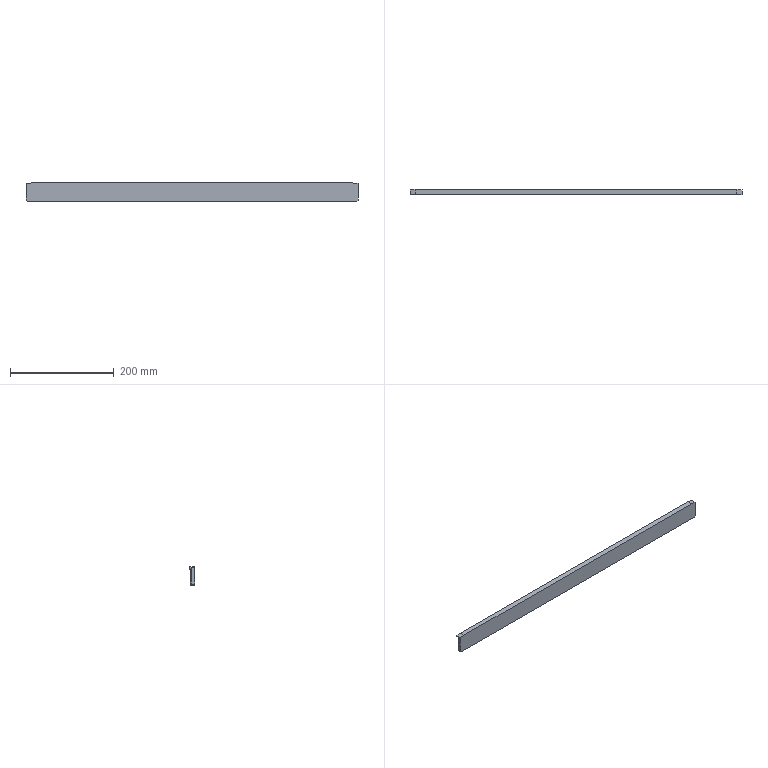Component | SolidWorks | XT-1-04-2-1 | 1 solid | 40 faces | box 640 x 10 x 35 mm | volume 184177 mm3 | plane 20 | cylinder 10 | cone 10 | commonest cylinder face diameters 3.3 x10
STEP:
#1=COLOUR_RGB('',0.7922,0.8196,0.9333);
#2=FILL_AREA_STYLE_COLOUR('',#1);
#3=FILL_AREA_STYLE('',(#2));
#4=SURFACE_STYLE_FILL_AREA(#3);
#5=SURFACE_SIDE_STYLE('',(#4));
#6=SURFACE_STYLE_USAGE(.BOTH.,#5);
#7=PRESENTATION_STYLE_ASSIGNMENT((#6));
#8=CARTESIAN_POINT('',(34.289,4.936,-5.035));
#9=VERTEX_POINT('',#8);
#10=CARTESIAN_POINT('',(34.159,4.936,-5.035));
#11=VERTEX_POINT('',#10);
#12=CARTESIAN_POINT('',(34.224,4.936,-5.035));
#13=DIRECTION('',(0.,0.,-1.));
#14=DIRECTION('',(-1.,0.,0.));
#15=AXIS2_PLACEMENT_3D('',#12,#13,#14);
#16=CIRCLE('',#15,0.06496);
#17=EDGE_CURVE('',#9,#11,#16,.T.);
#18=ORIENTED_EDGE('',*,*,#17,.F.);
#19=CARTESIAN_POINT('',(34.289,4.936,-5.433));
#20=VERTEX_POINT('',#19);
#21=CARTESIAN_POINT('',(34.289,4.936,-5.433));
#22=DIRECTION('',(0.,0.,-1.));
#23=VECTOR('',#22,39.37);
#24=LINE('',#21,#23);
#25=EDGE_CURVE('',#9,#20,#24,.T.);
#26=ORIENTED_EDGE('',*,*,#25,.T.);
#27=CARTESIAN_POINT('',(34.159,4.936,-5.433));
#28=VERTEX_POINT('',#27);
#29=CARTESIAN_POINT('',(34.224,4.936,-5.433));
#30=DIRECTION('',(0.,0.,-1.));
#31=DIRECTION('',(-1.,0.,0.));
#32=AXIS2_PLACEMENT_3D('',#29,#30,#31);
#33=CIRCLE('',#32,0.06496);
#34=EDGE_CURVE('',#20,#28,#33,.T.);
#35=ORIENTED_EDGE('',*,*,#34,.T.);
#36=CARTESIAN_POINT('',(34.159,4.936,-5.433));
#37=DIRECTION('',(0.,0.,-1.));
#38=VECTOR('',#37,39.37);
#39=LINE('',#36,#38);
#40=EDGE_CURVE('',#11,#28,#39,.T.);
#41=ORIENTED_EDGE('',*,*,#40,.F.);
#42=EDGE_LOOP('',(#18,#26,#35,#41));
#43=FACE_OUTER_BOUND('',#42,.T.);
#44=CARTESIAN_POINT('',(34.224,4.936,-5.433));
#45=DIRECTION('',(0.,0.,-1.));
#46=DIRECTION('',(-1.,0.,0.));
#47=AXIS2_PLACEMENT_3D('',#44,#45,#46);
#48=CYLINDRICAL_SURFACE('',#47,0.06496);
#49=ADVANCED_FACE('',(#43),#48,.F.);
#50=CARTESIAN_POINT('',(34.224,4.936,-4.996));
#51=VERTEX_POINT('',#50);
#52=CARTESIAN_POINT('',(34.159,4.936,-5.035));
#53=DIRECTION('',(-0.8572,0.,-0.515));
#54=VECTOR('',#53,39.37);
#55=LINE('',#52,#54);
#56=EDGE_CURVE('',#51,#11,#55,.T.);
#57=ORIENTED_EDGE('',*,*,#56,.F.);
#58=CARTESIAN_POINT('',(34.289,4.936,-5.035));
#59=DIRECTION('',(0.8572,0.,-0.515));
#60=VECTOR('',#59,39.37);
#61=LINE('',#58,#60);
#62=EDGE_CURVE('',#51,#9,#61,.T.);
#63=ORIENTED_EDGE('',*,*,#62,.T.);
#64=ORIENTED_EDGE('',*,*,#17,.T.);
#65=EDGE_LOOP('',(#57,#63,#64));
#66=FACE_OUTER_BOUND('',#65,.T.);
#67=CARTESIAN_POINT('',(34.224,4.936,-5.035));
#68=DIRECTION('',(0.,0.,-1.));
#69=DIRECTION('',(-1.,0.,0.));
#70=AXIS2_PLACEMENT_3D('',#67,#68,#69);
#71=CONICAL_SURFACE('',#70,0.06496,1.03);
#72=ADVANCED_FACE('',(#66),#71,.F.);
#73=CARTESIAN_POINT('',(28.777,4.936,-5.035));
#74=VERTEX_POINT('',#73);
#75=CARTESIAN_POINT('',(28.647,4.936,-5.035));
#76=VERTEX_POINT('',#75);
#77=CARTESIAN_POINT('',(28.712,4.936,-5.035));
#78=DIRECTION('',(0.,0.,-1.));
#79=DIRECTION('',(-1.,0.,0.));
#80=AXIS2_PLACEMENT_3D('',#77,#78,#79);
#81=CIRCLE('',#80,0.06496);
#82=EDGE_CURVE('',#74,#76,#81,.T.);
#83=ORIENTED_EDGE('',*,*,#82,.F.);
#84=CARTESIAN_POINT('',(28.777,4.936,-5.433));
#85=VERTEX_POINT('',#84);
#86=CARTESIAN_POINT('',(28.777,4.936,-5.433));
#87=DIRECTION('',(0.,0.,-1.));
#88=VECTOR('',#87,39.37);
#89=LINE('',#86,#88);
#90=EDGE_CURVE('',#74,#85,#89,.T.);
#91=ORIENTED_EDGE('',*,*,#90,.T.);
#92=CARTESIAN_POINT('',(28.647,4.936,-5.433));
#93=VERTEX_POINT('',#92);
#94=CARTESIAN_POINT('',(28.712,4.936,-5.433));
#95=DIRECTION('',(0.,0.,-1.));
#96=DIRECTION('',(-1.,0.,0.));
#97=AXIS2_PLACEMENT_3D('',#94,#95,#96);
#98=CIRCLE('',#97,0.06496);
#99=EDGE_CURVE('',#85,#93,#98,.T.);
#100=ORIENTED_EDGE('',*,*,#99,.T.);
#101=CARTESIAN_POINT('',(28.647,4.936,-5.433));
#102=DIRECTION('',(0.,0.,-1.));
#103=VECTOR('',#102,39.37);
#104=LINE('',#101,#103);
#105=EDGE_CURVE('',#76,#93,#104,.T.);
#106=ORIENTED_EDGE('',*,*,#105,.F.);
#107=EDGE_LOOP('',(#83,#91,#100,#106));
#108=FACE_OUTER_BOUND('',#107,.T.);
#109=CARTESIAN_POINT('',(28.712,4.936,-5.433));
#110=DIRECTION('',(0.,0.,-1.));
#111=DIRECTION('',(-1.,0.,0.));
#112=AXIS2_PLACEMENT_3D('',#109,#110,#111);
#113=CYLINDRICAL_SURFACE('',#112,0.06496);
#114=ADVANCED_FACE('',(#108),#113,.F.);
#115=CARTESIAN_POINT('',(28.712,4.936,-4.996));
#116=VERTEX_POINT('',#115);
#117=CARTESIAN_POINT('',(28.647,4.936,-5.035));
#118=DIRECTION('',(-0.8572,0.,-0.515));
#119=VECTOR('',#118,39.37);
#120=LINE('',#117,#119);
#121=EDGE_CURVE('',#116,#76,#120,.T.);
#122=ORIENTED_EDGE('',*,*,#121,.F.);
#123=CARTESIAN_POINT('',(28.777,4.936,-5.035));
#124=DIRECTION('',(0.8572,0.,-0.515));
#125=VECTOR('',#124,39.37);
#126=LINE('',#123,#125);
#127=EDGE_CURVE('',#116,#74,#126,.T.);
#128=ORIENTED_EDGE('',*,*,#127,.T.);
#129=ORIENTED_EDGE('',*,*,#82,.T.);
#130=EDGE_LOOP('',(#122,#128,#129));
#131=FACE_OUTER_BOUND('',#130,.T.);
#132=CARTESIAN_POINT('',(28.712,4.936,-5.035));
#133=DIRECTION('',(0.,0.,-1.));
#134=DIRECTION('',(-1.,0.,0.));
#135=AXIS2_PLACEMENT_3D('',#132,#133,#134);
#136=CONICAL_SURFACE('',#135,0.06496,1.03);
#137=ADVANCED_FACE('',(#131),#136,.F.);
#138=CARTESIAN_POINT('',(23.265,4.936,-5.035));
#139=VERTEX_POINT('',#138);
#140=CARTESIAN_POINT('',(23.135,4.936,-5.035));
#141=VERTEX_POINT('',#140);
#142=CARTESIAN_POINT('',(23.2,4.936,-5.035));
#143=DIRECTION('',(0.,0.,-1.));
#144=DIRECTION('',(-1.,0.,0.));
#145=AXIS2_PLACEMENT_3D('',#142,#143,#144);
#146=CIRCLE('',#145,0.06496);
#147=EDGE_CURVE('',#139,#141,#146,.T.);
#148=ORIENTED_EDGE('',*,*,#147,.F.);
#149=CARTESIAN_POINT('',(23.265,4.936,-5.433));
#150=VERTEX_POINT('',#149);
#151=CARTESIAN_POINT('',(23.265,4.936,-5.433));
#152=DIRECTION('',(0.,0.,-1.));
#153=VECTOR('',#152,39.37);
#154=LINE('',#151,#153);
#155=EDGE_CURVE('',#139,#150,#154,.T.);
#156=ORIENTED_EDGE('',*,*,#155,.T.);
#157=CARTESIAN_POINT('',(23.135,4.936,-5.433));
#158=VERTEX_POINT('',#157);
#159=CARTESIAN_POINT('',(23.2,4.936,-5.433));
#160=DIRECTION('',(0.,0.,-1.));
#161=DIRECTION('',(-1.,0.,0.));
#162=AXIS2_PLACEMENT_3D('',#159,#160,#161);
#163=CIRCLE('',#162,0.06496);
#164=EDGE_CURVE('',#150,#158,#163,.T.);
#165=ORIENTED_EDGE('',*,*,#164,.T.);
#166=CARTESIAN_POINT('',(23.135,4.936,-5.433));
#167=DIRECTION('',(0.,0.,-1.));
#168=VECTOR('',#167,39.37);
#169=LINE('',#166,#168);
#170=EDGE_CURVE('',#141,#158,#169,.T.);
#171=ORIENTED_EDGE('',*,*,#170,.F.);
#172=EDGE_LOOP('',(#148,#156,#165,#171));
#173=FACE_OUTER_BOUND('',#172,.T.);
#174=CARTESIAN_POINT('',(23.2,4.936,-5.433));
#175=DIRECTION('',(0.,0.,-1.));
#176=DIRECTION('',(-1.,0.,0.));
#177=AXIS2_PLACEMENT_3D('',#174,#175,#176);
#178=CYLINDRICAL_SURFACE('',#177,0.06496);
#179=ADVANCED_FACE('',(#173),#178,.F.);
#180=CARTESIAN_POINT('',(23.2,4.936,-4.996));
#181=VERTEX_POINT('',#180);
#182=CARTESIAN_POINT('',(23.135,4.936,-5.035));
#183=DIRECTION('',(-0.8572,0.,-0.515));
#184=VECTOR('',#183,39.37);
#185=LINE('',#182,#184);
#186=EDGE_CURVE('',#181,#141,#185,.T.);
#187=ORIENTED_EDGE('',*,*,#186,.F.);
#188=CARTESIAN_POINT('',(23.265,4.936,-5.035));
#189=DIRECTION('',(0.8572,0.,-0.515));
#190=VECTOR('',#189,39.37);
#191=LINE('',#188,#190);
#192=EDGE_CURVE('',#181,#139,#191,.T.);
#193=ORIENTED_EDGE('',*,*,#192,.T.);
#194=ORIENTED_EDGE('',*,*,#147,.T.);
#195=EDGE_LOOP('',(#187,#193,#194));
#196=FACE_OUTER_BOUND('',#195,.T.);
#197=CARTESIAN_POINT('',(23.2,4.936,-5.035));
#198=DIRECTION('',(0.,0.,-1.));
#199=DIRECTION('',(-1.,0.,0.));
#200=AXIS2_PLACEMENT_3D('',#197,#198,#199);
#201=CONICAL_SURFACE('',#200,0.06496,1.03);
#202=ADVANCED_FACE('',(#196),#201,.F.);
#203=CARTESIAN_POINT('',(17.753,4.936,-5.035));
#204=VERTEX_POINT('',#203);
#205=CARTESIAN_POINT('',(17.623,4.936,-5.035));
#206=VERTEX_POINT('',#205);
#207=CARTESIAN_POINT('',(17.688,4.936,-5.035));
#208=DIRECTION('',(0.,0.,-1.));
#209=DIRECTION('',(-1.,0.,0.));
#210=AXIS2_PLACEMENT_3D('',#207,#208,#209);
#211=CIRCLE('',#210,0.06496);
#212=EDGE_CURVE('',#204,#206,#211,.T.);
#213=ORIENTED_EDGE('',*,*,#212,.F.);
#214=CARTESIAN_POINT('',(17.753,4.936,-5.433));
#215=VERTEX_POINT('',#214);
#216=CARTESIAN_POINT('',(17.753,4.936,-5.433));
#217=DIRECTION('',(0.,0.,-1.));
#218=VECTOR('',#217,39.37);
#219=LINE('',#216,#218);
#220=EDGE_CURVE('',#204,#215,#219,.T.);
#221=ORIENTED_EDGE('',*,*,#220,.T.);
#222=CARTESIAN_POINT('',(17.623,4.936,-5.433));
#223=VERTEX_POINT('',#222);
#224=CARTESIAN_POINT('',(17.688,4.936,-5.433));
#225=DIRECTION('',(0.,0.,-1.));
#226=DIRECTION('',(-1.,0.,0.));
#227=AXIS2_PLACEMENT_3D('',#224,#225,#226);
#228=CIRCLE('',#227,0.06496);
#229=EDGE_CURVE('',#215,#223,#228,.T.);
#230=ORIENTED_EDGE('',*,*,#229,.T.);
#231=CARTESIAN_POINT('',(17.623,4.936,-5.433));
#232=DIRECTION('',(0.,0.,-1.));
#233=VECTOR('',#232,39.37);
#234=LINE('',#231,#233);
#235=EDGE_CURVE('',#206,#223,#234,.T.);
#236=ORIENTED_EDGE('',*,*,#235,.F.);
#237=EDGE_LOOP('',(#213,#221,#230,#236));
#238=FACE_OUTER_BOUND('',#237,.T.);
#239=CARTESIAN_POINT('',(17.688,4.936,-5.433));
#240=DIRECTION('',(0.,0.,-1.));
#241=DIRECTION('',(-1.,0.,0.));
#242=AXIS2_PLACEMENT_3D('',#239,#240,#241);
#243=CYLINDRICAL_SURFACE('',#242,0.06496);
#244=ADVANCED_FACE('',(#238),#243,.F.);
#245=CARTESIAN_POINT('',(17.688,4.936,-4.996));
#246=VERTEX_POINT('',#245);
#247=CARTESIAN_POINT('',(17.623,4.936,-5.035));
#248=DIRECTION('',(-0.8572,0.,-0.515));
#249=VECTOR('',#248,39.37);
#250=LINE('',#247,#249);
#251=EDGE_CURVE('',#246,#206,#250,.T.);
#252=ORIENTED_EDGE('',*,*,#251,.F.);
#253=CARTESIAN_POINT('',(17.753,4.936,-5.035));
#254=DIRECTION('',(0.8572,0.,-0.515));
#255=VECTOR('',#254,39.37);
#256=LINE('',#253,#255);
#257=EDGE_CURVE('',#246,#204,#256,.T.);
#258=ORIENTED_EDGE('',*,*,#257,.T.);
#259=ORIENTED_EDGE('',*,*,#212,.T.);
#260=EDGE_LOOP('',(#252,#258,#259));
#261=FACE_OUTER_BOUND('',#260,.T.);
#262=CARTESIAN_POINT('',(17.688,4.936,-5.035));
#263=DIRECTION('',(0.,0.,-1.));
#264=DIRECTION('',(-1.,0.,0.));
#265=AXIS2_PLACEMENT_3D('',#262,#263,#264);
#266=CONICAL_SURFACE('',#265,0.06496,1.03);
#267=ADVANCED_FACE('',(#261),#266,.F.);
#268=CARTESIAN_POINT('',(12.241,4.936,-5.035));
#269=VERTEX_POINT('',#268);
#270=CARTESIAN_POINT('',(12.112,4.936,-5.035));
#271=VERTEX_POINT('',#270);
#272=CARTESIAN_POINT('',(12.177,4.936,-5.035));
#273=DIRECTION('',(0.,0.,-1.));
#274=DIRECTION('',(-1.,0.,0.));
#275=AXIS2_PLACEMENT_3D('',#272,#273,#274);
#276=CIRCLE('',#275,0.06496);
#277=EDGE_CURVE('',#269,#271,#276,.T.);
#278=ORIENTED_EDGE('',*,*,#277,.F.);
#279=CARTESIAN_POINT('',(12.241,4.936,-5.433));
#280=VERTEX_POINT('',#279);
#281=CARTESIAN_POINT('',(12.241,4.936,-5.433));
#282=DIRECTION('',(0.,0.,-1.));
#283=VECTOR('',#282,39.37);
#284=LINE('',#281,#283);
#285=EDGE_CURVE('',#269,#280,#284,.T.);
#286=ORIENTED_EDGE('',*,*,#285,.T.);
#287=CARTESIAN_POINT('',(12.112,4.936,-5.433));
#288=VERTEX_POINT('',#287);
#289=CARTESIAN_POINT('',(12.177,4.936,-5.433));
#290=DIRECTION('',(0.,0.,-1.));
#291=DIRECTION('',(-1.,0.,0.));
#292=AXIS2_PLACEMENT_3D('',#289,#290,#291);
#293=CIRCLE('',#292,0.06496);
#294=EDGE_CURVE('',#280,#288,#293,.T.);
#295=ORIENTED_EDGE('',*,*,#294,.T.);
#296=CARTESIAN_POINT('',(12.112,4.936,-5.433));
#297=DIRECTION('',(0.,0.,-1.));
#298=VECTOR('',#297,39.37);
#299=LINE('',#296,#298);
#300=EDGE_CURVE('',#271,#288,#299,.T.);
#301=ORIENTED_EDGE('',*,*,#300,.F.);
#302=EDGE_LOOP('',(#278,#286,#295,#301));
#303=FACE_OUTER_BOUND('',#302,.T.);
#304=CARTESIAN_POINT('',(12.177,4.936,-5.433));
#305=DIRECTION('',(0.,0.,-1.));
#306=DIRECTION('',(-1.,0.,0.));
#307=AXIS2_PLACEMENT_3D('',#304,#305,#306);
#308=CYLINDRICAL_SURFACE('',#307,0.06496);
#309=ADVANCED_FACE('',(#303),#308,.F.);
#310=CARTESIAN_POINT('',(12.177,4.936,-4.996));
#311=VERTEX_POINT('',#310);
#312=CARTESIAN_POINT('',(12.112,4.936,-5.035));
#313=DIRECTION('',(-0.8572,0.,-0.515));
#314=VECTOR('',#313,39.37);
#315=LINE('',#312,#314);
#316=EDGE_CURVE('',#311,#271,#315,.T.);
#317=ORIENTED_EDGE('',*,*,#316,.F.);
#318=CARTESIAN_POINT('',(12.241,4.936,-5.035));
#319=DIRECTION('',(0.8572,0.,-0.515));
#320=VECTOR('',#319,39.37);
#321=LINE('',#318,#320);
#322=EDGE_CURVE('',#311,#269,#321,.T.);
#323=ORIENTED_EDGE('',*,*,#322,.T.);
#324=ORIENTED_EDGE('',*,*,#277,.T.);
#325=EDGE_LOOP('',(#317,#323,#324));
#326=FACE_OUTER_BOUND('',#325,.T.);
#327=CARTESIAN_POINT('',(12.177,4.936,-5.035));
#328=DIRECTION('',(0.,0.,-1.));
#329=DIRECTION('',(-1.,0.,0.));
#330=AXIS2_PLACEMENT_3D('',#327,#328,#329);
#331=CONICAL_SURFACE('',#330,0.06496,1.03);
#332=ADVANCED_FACE('',(#326),#331,.F.);
#333=CARTESIAN_POINT('',(35.405,5.173,-4.232));
#334=VERTEX_POINT('',#333);
#335=CARTESIAN_POINT('',(10.995,5.173,-4.232));
#336=VERTEX_POINT('',#335);
#337=CARTESIAN_POINT('',(35.799,5.173,-4.232));
#338=DIRECTION('',(-1.,0.,0.));
#339=VECTOR('',#338,39.37);
#340=LINE('',#337,#339);
#341=EDGE_CURVE('',#334,#336,#340,.T.);
#342=ORIENTED_EDGE('',*,*,#341,.T.);
#343=CARTESIAN_POINT('',(10.995,5.173,-4.075));
#344=VERTEX_POINT('',#343);
#345=CARTESIAN_POINT('',(10.995,5.173,-4.252));
#346=DIRECTION('',(0.,-0.,1.));
#347=VECTOR('',#346,39.37);
#348=LINE('',#345,#347);
#349=EDGE_CURVE('',#336,#344,#348,.T.);
#350=ORIENTED_EDGE('',*,*,#349,.T.);
#351=CARTESIAN_POINT('',(35.405,5.173,-4.075));
#352=VERTEX_POINT('',#351);
#353=CARTESIAN_POINT('',(35.799,5.173,-4.075));
#354=DIRECTION('',(1.,0.,0.));
#355=VECTOR('',#354,39.37);
#356=LINE('',#353,#355);
#357=EDGE_CURVE('',#344,#352,#356,.T.);
#358=ORIENTED_EDGE('',*,*,#357,.T.);
#359=CARTESIAN_POINT('',(35.405,5.173,-4.173));
#360=DIRECTION('',(0.,0.,-1.));
#361=VECTOR('',#360,39.37);
#362=LINE('',#359,#361);
#363=EDGE_CURVE('',#352,#334,#362,.T.);
#364=ORIENTED_EDGE('',*,*,#363,.T.);
#365=EDGE_LOOP('',(#342,#350,#358,#364));
#366=FACE_OUTER_BOUND('',#365,.T.);
#367=CARTESIAN_POINT('',(35.799,5.173,-4.252));
#368=DIRECTION('',(0.,-1.,-0.));
#369=DIRECTION('',(0.,0.,-1.));
#370=AXIS2_PLACEMENT_3D('',#367,#368,#369);
#371=PLANE('',#370);
#372=ADVANCED_FACE('',(#366),#371,.F.);
#373=CARTESIAN_POINT('',(35.405,5.153,-4.055));
#374=VERTEX_POINT('',#373);
#375=CARTESIAN_POINT('',(10.995,5.153,-4.055));
#376=VERTEX_POINT('',#375);
#377=CARTESIAN_POINT('',(35.799,5.153,-4.055));
#378=DIRECTION('',(-1.,0.,0.));
#379=VECTOR('',#378,39.37);
#380=LINE('',#377,#379);
#381=EDGE_CURVE('',#374,#376,#380,.T.);
#382=ORIENTED_EDGE('',*,*,#381,.T.);
#383=CARTESIAN_POINT('',(10.995,4.779,-4.055));
#384=VERTEX_POINT('',#383);
#385=CARTESIAN_POINT('',(10.995,5.173,-4.055));
#386=DIRECTION('',(0.,-1.,-0.));
#387=VECTOR('',#386,39.37);
#388=LINE('',#385,#387);
#389=EDGE_CURVE('',#376,#384,#388,.T.);
#390=ORIENTED_EDGE('',*,*,#389,.T.);
#391=CARTESIAN_POINT('',(35.405,4.779,-4.055));
#392=VERTEX_POINT('',#391);
#393=CARTESIAN_POINT('',(35.799,4.779,-4.055));
#394=DIRECTION('',(-1.,0.,0.));
#395=VECTOR('',#394,39.37);
#396=LINE('',#393,#395);
#397=EDGE_CURVE('',#392,#384,#396,.T.);
#398=ORIENTED_EDGE('',*,*,#397,.F.);
#399=CARTESIAN_POINT('',(35.405,5.153,-4.055));
#400=DIRECTION('',(0.,1.,0.));
#401=VECTOR('',#400,39.37);
#402=LINE('',#399,#401);
#403=EDGE_CURVE('',#392,#374,#402,.T.);
#404=ORIENTED_EDGE('',*,*,#403,.T.);
#405=EDGE_LOOP('',(#382,#390,#398,#404));
#406=FACE_OUTER_BOUND('',#405,.T.);
#407=CARTESIAN_POINT('',(35.799,5.173,-4.055));
#408=DIRECTION('',(0.,0.,-1.));
#409=DIRECTION('',(0.,1.,0.));
#410=AXIS2_PLACEMENT_3D('',#407,#408,#409);
#411=PLANE('',#410);
#412=ADVANCED_FACE('',(#406),#411,.F.);
#413=ORIENTED_EDGE('',*,*,#397,.T.);
#414=CARTESIAN_POINT('',(10.602,4.779,-4.094));
#415=VERTEX_POINT('',#414);
#416=CARTESIAN_POINT('',(10.995,4.779,-4.055));
#417=DIRECTION('',(-0.995,0.,-0.0995));
#418=VECTOR('',#417,39.37);
#419=LINE('',#416,#418);
#420=EDGE_CURVE('',#384,#415,#419,.T.);
#421=ORIENTED_EDGE('',*,*,#420,.T.);
#422=CARTESIAN_POINT('',(10.602,4.779,-5.354));
#423=VERTEX_POINT('',#422);
#424=CARTESIAN_POINT('',(10.602,4.779,-4.055));
#425=DIRECTION('',(0.,0.,-1.));
#426=VECTOR('',#425,39.37);
#427=LINE('',#424,#426);
#428=EDGE_CURVE('',#415,#423,#427,.T.);
#429=ORIENTED_EDGE('',*,*,#428,.T.);
#430=CARTESIAN_POINT('',(10.68,4.779,-5.433));
#431=VERTEX_POINT('',#430);
#432=CARTESIAN_POINT('',(10.68,4.779,-5.433));
#433=DIRECTION('',(0.7071,0.,-0.7071));
#434=VECTOR('',#433,39.37);
#435=LINE('',#432,#434);
#436=EDGE_CURVE('',#423,#431,#435,.T.);
#437=ORIENTED_EDGE('',*,*,#436,.T.);
#438=CARTESIAN_POINT('',(35.72,4.779,-5.433));
#439=VERTEX_POINT('',#438);
#440=CARTESIAN_POINT('',(35.799,4.779,-5.433));
#441=DIRECTION('',(-1.,0.,0.));
#442=VECTOR('',#441,39.37);
#443=LINE('',#440,#442);
#444=EDGE_CURVE('',#439,#431,#443,.T.);
#445=ORIENTED_EDGE('',*,*,#444,.F.);
#446=CARTESIAN_POINT('',(35.799,4.779,-5.354));
#447=VERTEX_POINT('',#446);
#448=CARTESIAN_POINT('',(35.799,4.779,-5.354));
#449=DIRECTION('',(0.7071,-0.,0.7071));
#450=VECTOR('',#449,39.37);
#451=LINE('',#448,#450);
#452=EDGE_CURVE('',#439,#447,#451,.T.);
#453=ORIENTED_EDGE('',*,*,#452,.T.);
#454=CARTESIAN_POINT('',(35.799,4.779,-4.094));
#455=VERTEX_POINT('',#454);
#456=CARTESIAN_POINT('',(35.799,4.779,-4.055));
#457=DIRECTION('',(0.,0.,-1.));
#458=VECTOR('',#457,39.37);
#459=LINE('',#456,#458);
#460=EDGE_CURVE('',#455,#447,#459,.T.);
#461=ORIENTED_EDGE('',*,*,#460,.F.);
#462=CARTESIAN_POINT('',(35.799,4.779,-4.094));
#463=DIRECTION('',(-0.995,-0.,0.0995));
#464=VECTOR('',#463,39.37);
#465=LINE('',#462,#464);
#466=EDGE_CURVE('',#455,#392,#465,.T.);
#467=ORIENTED_EDGE('',*,*,#466,.T.);
#468=EDGE_LOOP('',(#413,#421,#429,#437,#445,#453,#461,#467));
#469=FACE_OUTER_BOUND('',#468,.T.);
#470=CARTESIAN_POINT('',(35.799,4.779,-4.055));
#471=DIRECTION('',(0.,1.,0.));
#472=DIRECTION('',(0.,-0.,1.));
#473=AXIS2_PLACEMENT_3D('',#470,#471,#472);
#474=PLANE('',#473);
#475=ADVANCED_FACE('',(#469),#474,.F.);
#476=CARTESIAN_POINT('',(34.224,4.936,-5.433));
#477=DIRECTION('',(0.,0.,-1.));
#478=DIRECTION('',(-1.,0.,0.));
#479=AXIS2_PLACEMENT_3D('',#476,#477,#478);
#480=CIRCLE('',#479,0.06496);
#481=EDGE_CURVE('',#28,#20,#480,.T.);
#482=ORIENTED_EDGE('',*,*,#481,.F.);
#483=ORIENTED_EDGE('',*,*,#34,.F.);
#484=EDGE_LOOP('',(#482,#483));
#485=FACE_BOUND('',#484,.T.);
#486=CARTESIAN_POINT('',(28.712,4.936,-5.433));
#487=DIRECTION('',(0.,0.,-1.));
#488=DIRECTION('',(-1.,0.,0.));
#489=AXIS2_PLACEMENT_3D('',#486,#487,#488);
#490=CIRCLE('',#489,0.06496);
#491=EDGE_CURVE('',#93,#85,#490,.T.);
#492=ORIENTED_EDGE('',*,*,#491,.F.);
#493=ORIENTED_EDGE('',*,*,#99,.F.);
#494=EDGE_LOOP('',(#492,#493));
#495=FACE_BOUND('',#494,.T.);
#496=CARTESIAN_POINT('',(23.2,4.936,-5.433));
#497=DIRECTION('',(0.,0.,-1.));
#498=DIRECTION('',(-1.,0.,0.));
#499=AXIS2_PLACEMENT_3D('',#496,#497,#498);
#500=CIRCLE('',#499,0.06496);
#501=EDGE_CURVE('',#158,#150,#500,.T.);
#502=ORIENTED_EDGE('',*,*,#501,.F.);
#503=ORIENTED_EDGE('',*,*,#164,.F.);
#504=EDGE_LOOP('',(#502,#503));
#505=FACE_BOUND('',#504,.T.);
#506=CARTESIAN_POINT('',(17.688,4.936,-5.433));
#507=DIRECTION('',(0.,0.,-1.));
#508=DIRECTION('',(-1.,0.,0.));
#509=AXIS2_PLACEMENT_3D('',#506,#507,#508);
#510=CIRCLE('',#509,0.06496);
#511=EDGE_CURVE('',#223,#215,#510,.T.);
#512=ORIENTED_EDGE('',*,*,#511,.F.);
#513=ORIENTED_EDGE('',*,*,#229,.F.);
#514=EDGE_LOOP('',(#512,#513));
#515=FACE_BOUND('',#514,.T.);
#516=CARTESIAN_POINT('',(12.177,4.936,-5.433));
#517=DIRECTION('',(0.,0.,-1.));
#518=DIRECTION('',(-1.,0.,0.));
#519=AXIS2_PLACEMENT_3D('',#516,#517,#518);
#520=CIRCLE('',#519,0.06496);
#521=EDGE_CURVE('',#288,#280,#520,.T.);
#522=ORIENTED_EDGE('',*,*,#521,.F.);
#523=ORIENTED_EDGE('',*,*,#294,.F.);
#524=EDGE_LOOP('',(#522,#523));
#525=FACE_BOUND('',#524,.T.);
#526=ORIENTED_EDGE('',*,*,#444,.T.);
#527=CARTESIAN_POINT('',(10.68,5.031,-5.433));
#528=VERTEX_POINT('',#527);
#529=CARTESIAN_POINT('',(10.68,4.779,-5.433));
#530=DIRECTION('',(0.,1.,0.));
#531=VECTOR('',#530,39.37);
#532=LINE('',#529,#531);
#533=EDGE_CURVE('',#431,#528,#532,.T.);
#534=ORIENTED_EDGE('',*,*,#533,.T.);
#535=CARTESIAN_POINT('',(10.995,5.094,-5.433));
#536=VERTEX_POINT('',#535);
#537=CARTESIAN_POINT('',(10.995,5.094,-5.433));
#538=DIRECTION('',(0.9806,0.1961,0.));
#539=VECTOR('',#538,39.37);
#540=LINE('',#537,#539);
#541=EDGE_CURVE('',#528,#536,#540,.T.);
#542=ORIENTED_EDGE('',*,*,#541,.T.);
#543=CARTESIAN_POINT('',(35.405,5.094,-5.433));
#544=VERTEX_POINT('',#543);
#545=CARTESIAN_POINT('',(35.799,5.094,-5.433));
#546=DIRECTION('',(-1.,0.,0.));
#547=VECTOR('',#546,39.37);
#548=LINE('',#545,#547);
#549=EDGE_CURVE('',#544,#536,#548,.T.);
#550=ORIENTED_EDGE('',*,*,#549,.F.);
#551=CARTESIAN_POINT('',(35.72,5.031,-5.433));
#552=VERTEX_POINT('',#551);
#553=CARTESIAN_POINT('',(35.799,5.015,-5.433));
#554=DIRECTION('',(0.9806,-0.1961,0.));
#555=VECTOR('',#554,39.37);
#556=LINE('',#553,#555);
#557=EDGE_CURVE('',#544,#552,#556,.T.);
#558=ORIENTED_EDGE('',*,*,#557,.T.);
#559=CARTESIAN_POINT('',(35.72,4.779,-5.433));
#560=DIRECTION('',(0.,-1.,0.));
#561=VECTOR('',#560,39.37);
#562=LINE('',#559,#561);
#563=EDGE_CURVE('',#552,#439,#562,.T.);
#564=ORIENTED_EDGE('',*,*,#563,.T.);
#565=EDGE_LOOP('',(#526,#534,#542,#550,#558,#564));
#566=FACE_OUTER_BOUND('',#565,.T.);
#567=CARTESIAN_POINT('',(35.799,4.779,-5.433));
#568=DIRECTION('',(0.,0.,1.));
#569=DIRECTION('',(1.,0.,0.));
#570=AXIS2_PLACEMENT_3D('',#567,#568,#569);
#571=PLANE('',#570);
#572=ADVANCED_FACE('',(#485,#495,#505,#515,#525,#566),#571,.F.);
#573=ORIENTED_EDGE('',*,*,#549,.T.);
#574=CARTESIAN_POINT('',(10.995,5.094,-4.252));
#575=VERTEX_POINT('',#574);
#576=CARTESIAN_POINT('',(10.995,5.094,-5.433));
#577=DIRECTION('',(0.,-0.,1.));
#578=VECTOR('',#577,39.37);
#579=LINE('',#576,#578);
#580=EDGE_CURVE('',#536,#575,#579,.T.);
#581=ORIENTED_EDGE('',*,*,#580,.T.);
#582=CARTESIAN_POINT('',(35.405,5.094,-4.252));
#583=VERTEX_POINT('',#582);
#584=CARTESIAN_POINT('',(35.799,5.094,-4.252));
#585=DIRECTION('',(-1.,0.,0.));
#586=VECTOR('',#585,39.37);
#587=LINE('',#584,#586);
#588=EDGE_CURVE('',#583,#575,#587,.T.);
#589=ORIENTED_EDGE('',*,*,#588,.F.);
#590=CARTESIAN_POINT('',(35.405,5.094,-5.433));
#591=DIRECTION('',(0.,0.,-1.));
#592=VECTOR('',#591,39.37);
#593=LINE('',#590,#592);
#594=EDGE_CURVE('',#583,#544,#593,.T.);
#595=ORIENTED_EDGE('',*,*,#594,.T.);
#596=EDGE_LOOP('',(#573,#581,#589,#595));
#597=FACE_OUTER_BOUND('',#596,.T.);
#598=CARTESIAN_POINT('',(35.799,5.094,-5.433));
#599=DIRECTION('',(0.,-1.,-0.));
#600=DIRECTION('',(0.,0.,-1.));
#601=AXIS2_PLACEMENT_3D('',#598,#599,#600);
#602=PLANE('',#601);
#603=ADVANCED_FACE('',(#597),#602,.F.);
#604=CARTESIAN_POINT('',(10.995,5.153,-4.252));
#605=VERTEX_POINT('',#604);
#606=CARTESIAN_POINT('',(10.995,5.094,-4.252));
#607=DIRECTION('',(0.,1.,0.));
#608=VECTOR('',#607,39.37);
#609=LINE('',#606,#608);
#610=EDGE_CURVE('',#575,#605,#609,.T.);
#611=ORIENTED_EDGE('',*,*,#610,.T.);
#612=CARTESIAN_POINT('',(35.405,5.153,-4.252));
#613=VERTEX_POINT('',#612);
#614=CARTESIAN_POINT('',(35.799,5.153,-4.252));
#615=DIRECTION('',(1.,0.,0.));
#616=VECTOR('',#615,39.37);
#617=LINE('',#614,#616);
#618=EDGE_CURVE('',#605,#613,#617,.T.);
#619=ORIENTED_EDGE('',*,*,#618,.T.);
#620=CARTESIAN_POINT('',(35.405,5.094,-4.252));
#621=DIRECTION('',(0.,-1.,0.));
#622=VECTOR('',#621,39.37);
#623=LINE('',#620,#622);
#624=EDGE_CURVE('',#613,#583,#623,.T.);
#625=ORIENTED_EDGE('',*,*,#624,.T.);
#626=ORIENTED_EDGE('',*,*,#588,.T.);
#627=EDGE_LOOP('',(#611,#619,#625,#626));
#628=FACE_OUTER_BOUND('',#627,.T.);
#629=CARTESIAN_POINT('',(35.799,5.094,-4.252));
#630=DIRECTION('',(0.,0.,1.));
#631=DIRECTION('',(1.,0.,0.));
#632=AXIS2_PLACEMENT_3D('',#629,#630,#631);
#633=PLANE('',#632);
#634=ADVANCED_FACE('',(#628),#633,.F.);
#635=CARTESIAN_POINT('',(35.799,5.015,-4.173));
#636=VERTEX_POINT('',#635);
#637=CARTESIAN_POINT('',(35.799,5.133,-4.173));
#638=VERTEX_POINT('',#637);
#639=CARTESIAN_POINT('',(35.799,5.173,-4.173));
#640=DIRECTION('',(0.,1.,0.));
#641=VECTOR('',#640,39.37);
#642=LINE('',#639,#641);
#643=EDGE_CURVE('',#636,#638,#642,.T.);
#644=ORIENTED_EDGE('',*,*,#643,.T.);
#645=CARTESIAN_POINT('',(35.799,5.133,-4.094));
#646=VERTEX_POINT('',#645);
#647=CARTESIAN_POINT('',(35.799,5.133,-4.094));
#648=DIRECTION('',(0.,-0.,1.));
#649=VECTOR('',#648,39.37);
#650=LINE('',#647,#649);
#651=EDGE_CURVE('',#638,#646,#650,.T.);
#652=ORIENTED_EDGE('',*,*,#651,.T.);
#653=CARTESIAN_POINT('',(35.799,4.779,-4.094));
#654=DIRECTION('',(0.,-1.,-0.));
#655=VECTOR('',#654,39.37);
#656=LINE('',#653,#655);
#657=EDGE_CURVE('',#646,#455,#656,.T.);
#658=ORIENTED_EDGE('',*,*,#657,.T.);
#659=ORIENTED_EDGE('',*,*,#460,.T.);
#660=CARTESIAN_POINT('',(35.799,5.015,-5.354));
#661=VERTEX_POINT('',#660);
#662=CARTESIAN_POINT('',(35.799,5.015,-5.354));
#663=DIRECTION('',(0.,1.,0.));
#664=VECTOR('',#663,39.37);
#665=LINE('',#662,#664);
#666=EDGE_CURVE('',#447,#661,#665,.T.);
#667=ORIENTED_EDGE('',*,*,#666,.T.);
#668=CARTESIAN_POINT('',(35.799,5.015,-4.252));
#669=DIRECTION('',(0.,-0.,1.));
#670=VECTOR('',#669,39.37);
#671=LINE('',#668,#670);
#672=EDGE_CURVE('',#661,#636,#671,.T.);
#673=ORIENTED_EDGE('',*,*,#672,.T.);
#674=EDGE_LOOP('',(#644,#652,#658,#659,#667,#673));
#675=FACE_OUTER_BOUND('',#674,.T.);
#676=CARTESIAN_POINT('',(35.799,5.173,-4.055));
#677=DIRECTION('',(1.,0.,0.));
#678=DIRECTION('',(0.,0.,-1.));
#679=AXIS2_PLACEMENT_3D('',#676,#677,#678);
#680=PLANE('',#679);
#681=ADVANCED_FACE('',(#675),#680,.T.);
#682=CARTESIAN_POINT('',(10.602,5.133,-4.094));
#683=VERTEX_POINT('',#682);
#684=CARTESIAN_POINT('',(10.602,5.173,-4.094));
#685=DIRECTION('',(0.,1.,0.));
#686=VECTOR('',#685,39.37);
#687=LINE('',#684,#686);
#688=EDGE_CURVE('',#415,#683,#687,.T.);
#689=ORIENTED_EDGE('',*,*,#688,.T.);
#690=CARTESIAN_POINT('',(10.602,5.133,-4.173));
#691=VERTEX_POINT('',#690);
#692=CARTESIAN_POINT('',(10.602,5.133,-4.055));
#693=DIRECTION('',(0.,0.,-1.));
#694=VECTOR('',#693,39.37);
#695=LINE('',#692,#694);
#696=EDGE_CURVE('',#683,#691,#695,.T.);
#697=ORIENTED_EDGE('',*,*,#696,.T.);
#698=CARTESIAN_POINT('',(10.602,5.015,-4.173));
#699=VERTEX_POINT('',#698);
#700=CARTESIAN_POINT('',(10.602,5.173,-4.173));
#701=DIRECTION('',(0.,-1.,0.));
#702=VECTOR('',#701,39.37);
#703=LINE('',#700,#702);
#704=EDGE_CURVE('',#691,#699,#703,.T.);
#705=ORIENTED_EDGE('',*,*,#704,.T.);
#706=CARTESIAN_POINT('',(10.602,5.015,-5.354));
#707=VERTEX_POINT('',#706);
#708=CARTESIAN_POINT('',(10.602,5.015,-4.055));
#709=DIRECTION('',(0.,0.,-1.));
#710=VECTOR('',#709,39.37);
#711=LINE('',#708,#710);
#712=EDGE_CURVE('',#699,#707,#711,.T.);
#713=ORIENTED_EDGE('',*,*,#712,.T.);
#714=CARTESIAN_POINT('',(10.602,5.173,-5.354));
#715=DIRECTION('',(0.,-1.,0.));
#716=VECTOR('',#715,39.37);
#717=LINE('',#714,#716);
#718=EDGE_CURVE('',#707,#423,#717,.T.);
#719=ORIENTED_EDGE('',*,*,#718,.T.);
#720=ORIENTED_EDGE('',*,*,#428,.F.);
#721=EDGE_LOOP('',(#689,#697,#705,#713,#719,#720));
#722=FACE_OUTER_BOUND('',#721,.T.);
#723=CARTESIAN_POINT('',(10.602,5.173,-4.055));
#724=DIRECTION('',(1.,0.,0.));
#725=DIRECTION('',(0.,0.,-1.));
#726=AXIS2_PLACEMENT_3D('',#723,#724,#725);
#727=PLANE('',#726);
#728=ADVANCED_FACE('',(#722),#727,.F.);
#729=ORIENTED_EDGE('',*,*,#322,.F.);
#730=ORIENTED_EDGE('',*,*,#316,.T.);
#731=CARTESIAN_POINT('',(12.177,4.936,-5.035));
#732=DIRECTION('',(0.,0.,-1.));
#733=DIRECTION('',(-1.,0.,0.));
#734=AXIS2_PLACEMENT_3D('',#731,#732,#733);
#735=CIRCLE('',#734,0.06496);
#736=EDGE_CURVE('',#271,#269,#735,.T.);
#737=ORIENTED_EDGE('',*,*,#736,.T.);
#738=EDGE_LOOP('',(#729,#730,#737));
#739=FACE_OUTER_BOUND('',#738,.T.);
#740=CARTESIAN_POINT('',(12.177,4.936,-5.035));
#741=DIRECTION('',(0.,0.,-1.));
#742=DIRECTION('',(-1.,0.,0.));
#743=AXIS2_PLACEMENT_3D('',#740,#741,#742);
#744=CONICAL_SURFACE('',#743,0.06496,1.03);
#745=ADVANCED_FACE('',(#739),#744,.F.);
#746=ORIENTED_EDGE('',*,*,#285,.F.);
#747=ORIENTED_EDGE('',*,*,#736,.F.);
#748=ORIENTED_EDGE('',*,*,#300,.T.);
#749=ORIENTED_EDGE('',*,*,#521,.T.);
#750=EDGE_LOOP('',(#746,#747,#748,#749));
#751=FACE_OUTER_BOUND('',#750,.T.);
#752=CARTESIAN_POINT('',(12.177,4.936,-5.433));
#753=DIRECTION('',(0.,0.,-1.));
#754=DIRECTION('',(-1.,0.,0.));
#755=AXIS2_PLACEMENT_3D('',#752,#753,#754);
#756=CYLINDRICAL_SURFACE('',#755,0.06496);
#757=ADVANCED_FACE('',(#751),#756,.F.);
#758=ORIENTED_EDGE('',*,*,#257,.F.);
#759=ORIENTED_EDGE('',*,*,#251,.T.);
#760=CARTESIAN_POINT('',(17.688,4.936,-5.035));
#761=DIRECTION('',(0.,0.,-1.));
#762=DIRECTION('',(-1.,0.,0.));
#763=AXIS2_PLACEMENT_3D('',#760,#761,#762);
#764=CIRCLE('',#763,0.06496);
#765=EDGE_CURVE('',#206,#204,#764,.T.);
#766=ORIENTED_EDGE('',*,*,#765,.T.);
#767=EDGE_LOOP('',(#758,#759,#766));
#768=FACE_OUTER_BOUND('',#767,.T.);
#769=CARTESIAN_POINT('',(17.688,4.936,-5.035));
#770=DIRECTION('',(0.,0.,-1.));
#771=DIRECTION('',(-1.,0.,0.));
#772=AXIS2_PLACEMENT_3D('',#769,#770,#771);
#773=CONICAL_SURFACE('',#772,0.06496,1.03);
#774=ADVANCED_FACE('',(#768),#773,.F.);
#775=ORIENTED_EDGE('',*,*,#220,.F.);
#776=ORIENTED_EDGE('',*,*,#765,.F.);
#777=ORIENTED_EDGE('',*,*,#235,.T.);
#778=ORIENTED_EDGE('',*,*,#511,.T.);
#779=EDGE_LOOP('',(#775,#776,#777,#778));
#780=FACE_OUTER_BOUND('',#779,.T.);
#781=CARTESIAN_POINT('',(17.688,4.936,-5.433));
#782=DIRECTION('',(0.,0.,-1.));
#783=DIRECTION('',(-1.,0.,0.));
#784=AXIS2_PLACEMENT_3D('',#781,#782,#783);
#785=CYLINDRICAL_SURFACE('',#784,0.06496);
#786=ADVANCED_FACE('',(#780),#785,.F.);
#787=ORIENTED_EDGE('',*,*,#192,.F.);
#788=ORIENTED_EDGE('',*,*,#186,.T.);
#789=CARTESIAN_POINT('',(23.2,4.936,-5.035));
#790=DIRECTION('',(0.,0.,-1.));
#791=DIRECTION('',(-1.,0.,0.));
#792=AXIS2_PLACEMENT_3D('',#789,#790,#791);
#793=CIRCLE('',#792,0.06496);
#794=EDGE_CURVE('',#141,#139,#793,.T.);
#795=ORIENTED_EDGE('',*,*,#794,.T.);
#796=EDGE_LOOP('',(#787,#788,#795));
#797=FACE_OUTER_BOUND('',#796,.T.);
#798=CARTESIAN_POINT('',(23.2,4.936,-5.035));
#799=DIRECTION('',(0.,0.,-1.));
#800=DIRECTION('',(-1.,0.,0.));
#801=AXIS2_PLACEMENT_3D('',#798,#799,#800);
#802=CONICAL_SURFACE('',#801,0.06496,1.03);
#803=ADVANCED_FACE('',(#797),#802,.F.);
#804=ORIENTED_EDGE('',*,*,#155,.F.);
#805=ORIENTED_EDGE('',*,*,#794,.F.);
#806=ORIENTED_EDGE('',*,*,#170,.T.);
#807=ORIENTED_EDGE('',*,*,#501,.T.);
#808=EDGE_LOOP('',(#804,#805,#806,#807));
#809=FACE_OUTER_BOUND('',#808,.T.);
#810=CARTESIAN_POINT('',(23.2,4.936,-5.433));
#811=DIRECTION('',(0.,0.,-1.));
#812=DIRECTION('',(-1.,0.,0.));
#813=AXIS2_PLACEMENT_3D('',#810,#811,#812);
#814=CYLINDRICAL_SURFACE('',#813,0.06496);
#815=ADVANCED_FACE('',(#809),#814,.F.);
#816=ORIENTED_EDGE('',*,*,#127,.F.);
#817=ORIENTED_EDGE('',*,*,#121,.T.);
#818=CARTESIAN_POINT('',(28.712,4.936,-5.035));
#819=DIRECTION('',(0.,0.,-1.));
#820=DIRECTION('',(-1.,0.,0.));
#821=AXIS2_PLACEMENT_3D('',#818,#819,#820);
#822=CIRCLE('',#821,0.06496);
#823=EDGE_CURVE('',#76,#74,#822,.T.);
#824=ORIENTED_EDGE('',*,*,#823,.T.);
#825=EDGE_LOOP('',(#816,#817,#824));
#826=FACE_OUTER_BOUND('',#825,.T.);
#827=CARTESIAN_POINT('',(28.712,4.936,-5.035));
#828=DIRECTION('',(0.,0.,-1.));
#829=DIRECTION('',(-1.,0.,0.));
#830=AXIS2_PLACEMENT_3D('',#827,#828,#829);
#831=CONICAL_SURFACE('',#830,0.06496,1.03);
#832=ADVANCED_FACE('',(#826),#831,.F.);
#833=ORIENTED_EDGE('',*,*,#90,.F.);
#834=ORIENTED_EDGE('',*,*,#823,.F.);
#835=ORIENTED_EDGE('',*,*,#105,.T.);
#836=ORIENTED_EDGE('',*,*,#491,.T.);
#837=EDGE_LOOP('',(#833,#834,#835,#836));
#838=FACE_OUTER_BOUND('',#837,.T.);
#839=CARTESIAN_POINT('',(28.712,4.936,-5.433));
#840=DIRECTION('',(0.,0.,-1.));
#841=DIRECTION('',(-1.,0.,0.));
#842=AXIS2_PLACEMENT_3D('',#839,#840,#841);
#843=CYLINDRICAL_SURFACE('',#842,0.06496);
#844=ADVANCED_FACE('',(#838),#843,.F.);
#845=ORIENTED_EDGE('',*,*,#62,.F.);
#846=ORIENTED_EDGE('',*,*,#56,.T.);
#847=CARTESIAN_POINT('',(34.224,4.936,-5.035));
#848=DIRECTION('',(0.,0.,-1.));
#849=DIRECTION('',(-1.,0.,0.));
#850=AXIS2_PLACEMENT_3D('',#847,#848,#849);
#851=CIRCLE('',#850,0.06496);
#852=EDGE_CURVE('',#11,#9,#851,.T.);
#853=ORIENTED_EDGE('',*,*,#852,.T.);
#854=EDGE_LOOP('',(#845,#846,#853));
#855=FACE_OUTER_BOUND('',#854,.T.);
#856=CARTESIAN_POINT('',(34.224,4.936,-5.035));
#857=DIRECTION('',(0.,0.,-1.));
#858=DIRECTION('',(-1.,0.,0.));
#859=AXIS2_PLACEMENT_3D('',#856,#857,#858);
#860=CONICAL_SURFACE('',#859,0.06496,1.03);
#861=ADVANCED_FACE('',(#855),#860,.F.);
#862=ORIENTED_EDGE('',*,*,#25,.F.);
#863=ORIENTED_EDGE('',*,*,#852,.F.);
#864=ORIENTED_EDGE('',*,*,#40,.T.);
#865=ORIENTED_EDGE('',*,*,#481,.T.);
#866=EDGE_LOOP('',(#862,#863,#864,#865));
#867=FACE_OUTER_BOUND('',#866,.T.);
#868=CARTESIAN_POINT('',(34.224,4.936,-5.433));
#869=DIRECTION('',(0.,0.,-1.));
#870=DIRECTION('',(-1.,0.,0.));
#871=AXIS2_PLACEMENT_3D('',#868,#869,#870);
#872=CYLINDRICAL_SURFACE('',#871,0.06496);
#873=ADVANCED_FACE('',(#867),#872,.F.);
#874=ORIENTED_EDGE('',*,*,#704,.F.);
#875=CARTESIAN_POINT('',(10.93,5.166,-4.239));
#876=VERTEX_POINT('',#875);
#877=CARTESIAN_POINT('',(10.988,5.172,-4.25));
#878=DIRECTION('',(0.9759,0.09759,-0.1952));
#879=VECTOR('',#878,39.37);
#880=LINE('',#877,#879);
#881=EDGE_CURVE('',#691,#876,#880,.T.);
#882=ORIENTED_EDGE('',*,*,#881,.T.);
#883=CARTESIAN_POINT('',(11.006,5.151,-4.254));
#884=DIRECTION('',(0.9623,-0.1925,-0.1925));
#885=VECTOR('',#884,39.37);
#886=LINE('',#883,#885);
#887=EDGE_CURVE('',#876,#605,#886,.T.);
#888=ORIENTED_EDGE('',*,*,#887,.T.);
#889=ORIENTED_EDGE('',*,*,#610,.F.);
#890=CARTESIAN_POINT('',(11.214,5.138,-4.296));
#891=DIRECTION('',(0.9623,0.1925,-0.1925));
#892=VECTOR('',#891,39.37);
#893=LINE('',#890,#892);
#894=EDGE_CURVE('',#699,#575,#893,.T.);
#895=ORIENTED_EDGE('',*,*,#894,.F.);
#896=EDGE_LOOP('',(#874,#882,#888,#889,#895));
#897=FACE_OUTER_BOUND('',#896,.T.);
#898=CARTESIAN_POINT('',(10.995,5.094,-4.252));
#899=DIRECTION('',(0.1961,0.,0.9806));
#900=DIRECTION('',(0.,1.,0.));
#901=AXIS2_PLACEMENT_3D('',#898,#899,#900);
#902=PLANE('',#901);
#903=ADVANCED_FACE('',(#897),#902,.F.);
#904=ORIENTED_EDGE('',*,*,#541,.F.);
#905=CARTESIAN_POINT('',(10.841,5.063,-5.594));
#906=DIRECTION('',(-0.7001,-0.14,0.7001));
#907=VECTOR('',#906,39.37);
#908=LINE('',#905,#907);
#909=EDGE_CURVE('',#528,#707,#908,.T.);
#910=ORIENTED_EDGE('',*,*,#909,.T.);
#911=ORIENTED_EDGE('',*,*,#712,.F.);
#912=ORIENTED_EDGE('',*,*,#894,.T.);
#913=ORIENTED_EDGE('',*,*,#580,.F.);
#914=EDGE_LOOP('',(#904,#910,#911,#912,#913));
#915=FACE_OUTER_BOUND('',#914,.T.);
#916=CARTESIAN_POINT('',(10.995,5.094,-5.433));
#917=DIRECTION('',(0.1961,-0.9806,-0.));
#918=DIRECTION('',(0.,-0.,1.));
#919=AXIS2_PLACEMENT_3D('',#916,#917,#918);
#920=PLANE('',#919);
#921=ADVANCED_FACE('',(#915),#920,.F.);
#922=CARTESIAN_POINT('',(35.47,5.166,-4.239));
#923=VERTEX_POINT('',#922);
#924=CARTESIAN_POINT('',(35.788,5.23,-4.175));
#925=DIRECTION('',(0.9623,0.1925,0.1925));
#926=VECTOR('',#925,39.37);
#927=LINE('',#924,#926);
#928=EDGE_CURVE('',#613,#923,#927,.T.);
#929=ORIENTED_EDGE('',*,*,#928,.T.);
#930=CARTESIAN_POINT('',(35.795,5.134,-4.174));
#931=DIRECTION('',(0.9759,-0.09759,0.1952));
#932=VECTOR('',#931,39.37);
#933=LINE('',#930,#932);
#934=EDGE_CURVE('',#923,#638,#933,.T.);
#935=ORIENTED_EDGE('',*,*,#934,.T.);
#936=ORIENTED_EDGE('',*,*,#643,.F.);
#937=CARTESIAN_POINT('',(35.82,5.011,-4.169));
#938=DIRECTION('',(0.9623,-0.1925,0.1925));
#939=VECTOR('',#938,39.37);
#940=LINE('',#937,#939);
#941=EDGE_CURVE('',#583,#636,#940,.T.);
#942=ORIENTED_EDGE('',*,*,#941,.F.);
#943=ORIENTED_EDGE('',*,*,#624,.F.);
#944=EDGE_LOOP('',(#929,#935,#936,#942,#943));
#945=FACE_OUTER_BOUND('',#944,.T.);
#946=CARTESIAN_POINT('',(35.799,5.173,-4.173));
#947=DIRECTION('',(0.1961,0.,-0.9806));
#948=DIRECTION('',(0.,-1.,0.));
#949=AXIS2_PLACEMENT_3D('',#946,#947,#948);
#950=PLANE('',#949);
#951=ADVANCED_FACE('',(#945),#950,.T.);
#952=ORIENTED_EDGE('',*,*,#672,.F.);
#953=CARTESIAN_POINT('',(36.435,4.888,-4.717));
#954=DIRECTION('',(-0.7001,0.14,-0.7001));
#955=VECTOR('',#954,39.37);
#956=LINE('',#953,#955);
#957=EDGE_CURVE('',#661,#552,#956,.T.);
#958=ORIENTED_EDGE('',*,*,#957,.T.);
#959=ORIENTED_EDGE('',*,*,#557,.F.);
#960=ORIENTED_EDGE('',*,*,#594,.F.);
#961=ORIENTED_EDGE('',*,*,#941,.T.);
#962=EDGE_LOOP('',(#952,#958,#959,#960,#961));
#963=FACE_OUTER_BOUND('',#962,.T.);
#964=CARTESIAN_POINT('',(35.799,5.015,-4.055));
#965=DIRECTION('',(0.1961,0.9806,0.));
#966=DIRECTION('',(0.,0.,-1.));
#967=AXIS2_PLACEMENT_3D('',#964,#965,#966);
#968=PLANE('',#967);
#969=ADVANCED_FACE('',(#963),#968,.T.);
#970=ORIENTED_EDGE('',*,*,#357,.F.);
#971=CARTESIAN_POINT('',(10.897,5.163,-4.065));
#972=VERTEX_POINT('',#971);
#973=CARTESIAN_POINT('',(35.308,7.604,-6.506));
#974=DIRECTION('',(-0.9901,-0.09901,0.09901));
#975=VECTOR('',#974,39.37);
#976=LINE('',#973,#975);
#977=EDGE_CURVE('',#344,#972,#976,.T.);
#978=ORIENTED_EDGE('',*,*,#977,.T.);
#979=CARTESIAN_POINT('',(35.312,2.721,-1.623));
#980=DIRECTION('',(0.9901,-0.09901,0.09901));
#981=VECTOR('',#980,39.37);
#982=LINE('',#979,#981);
#983=EDGE_CURVE('',#972,#376,#982,.T.);
#984=ORIENTED_EDGE('',*,*,#983,.T.);
#985=ORIENTED_EDGE('',*,*,#381,.F.);
#986=CARTESIAN_POINT('',(35.503,5.163,-4.065));
#987=VERTEX_POINT('',#986);
#988=CARTESIAN_POINT('',(35.791,5.192,-4.094));
#989=DIRECTION('',(0.9901,0.09901,-0.09901));
#990=VECTOR('',#989,39.37);
#991=LINE('',#988,#990);
#992=EDGE_CURVE('',#374,#987,#991,.T.);
#993=ORIENTED_EDGE('',*,*,#992,.T.);
#994=CARTESIAN_POINT('',(35.795,5.134,-4.036));
#995=DIRECTION('',(-0.9901,0.09901,-0.09901));
#996=VECTOR('',#995,39.37);
#997=LINE('',#994,#996);
#998=EDGE_CURVE('',#987,#352,#997,.T.);
#999=ORIENTED_EDGE('',*,*,#998,.T.);
#1000=EDGE_LOOP('',(#970,#978,#984,#985,#993,#999));
#1001=FACE_OUTER_BOUND('',#1000,.T.);
#1002=CARTESIAN_POINT('',(35.799,5.153,-4.055));
#1003=DIRECTION('',(0.,-0.7071,-0.7071));
#1004=DIRECTION('',(-1.,0.,0.));
#1005=AXIS2_PLACEMENT_3D('',#1002,#1003,#1004);
#1006=PLANE('',#1005);
#1007=ADVANCED_FACE('',(#1001),#1006,.F.);
#1008=ORIENTED_EDGE('',*,*,#887,.F.);
#1009=CARTESIAN_POINT('',(35.312,7.604,-1.801));
#1010=DIRECTION('',(0.9901,0.09901,0.09901));
#1011=VECTOR('',#1010,39.37);
#1012=LINE('',#1009,#1011);
#1013=EDGE_CURVE('',#876,#336,#1012,.T.);
#1014=ORIENTED_EDGE('',*,*,#1013,.T.);
#1015=ORIENTED_EDGE('',*,*,#341,.F.);
#1016=CARTESIAN_POINT('',(35.791,5.134,-4.271));
#1017=DIRECTION('',(0.9901,-0.09901,-0.09901));
#1018=VECTOR('',#1017,39.37);
#1019=LINE('',#1016,#1018);
#1020=EDGE_CURVE('',#334,#923,#1019,.T.);
#1021=ORIENTED_EDGE('',*,*,#1020,.T.);
#1022=ORIENTED_EDGE('',*,*,#928,.F.);
#1023=ORIENTED_EDGE('',*,*,#618,.F.);
#1024=EDGE_LOOP('',(#1008,#1014,#1015,#1021,#1022,#1023));
#1025=FACE_OUTER_BOUND('',#1024,.T.);
#1026=CARTESIAN_POINT('',(35.799,5.173,-4.232));
#1027=DIRECTION('',(0.,-0.7071,0.7071));
#1028=DIRECTION('',(-1.,0.,0.));
#1029=AXIS2_PLACEMENT_3D('',#1026,#1027,#1028);
#1030=PLANE('',#1029);
#1031=ADVANCED_FACE('',(#1025),#1030,.F.);
#1032=ORIENTED_EDGE('',*,*,#436,.F.);
#1033=ORIENTED_EDGE('',*,*,#718,.F.);
#1034=ORIENTED_EDGE('',*,*,#909,.F.);
#1035=ORIENTED_EDGE('',*,*,#533,.F.);
#1036=EDGE_LOOP('',(#1032,#1033,#1034,#1035));
#1037=FACE_OUTER_BOUND('',#1036,.T.);
#1038=CARTESIAN_POINT('',(10.68,4.779,-5.433));
#1039=DIRECTION('',(0.7071,0.,0.7071));
#1040=DIRECTION('',(0.,1.,0.));
#1041=AXIS2_PLACEMENT_3D('',#1038,#1039,#1040);
#1042=PLANE('',#1041);
#1043=ADVANCED_FACE('',(#1037),#1042,.F.);
#1044=ORIENTED_EDGE('',*,*,#452,.F.);
#1045=ORIENTED_EDGE('',*,*,#563,.F.);
#1046=ORIENTED_EDGE('',*,*,#957,.F.);
#1047=ORIENTED_EDGE('',*,*,#666,.F.);
#1048=EDGE_LOOP('',(#1044,#1045,#1046,#1047));
#1049=FACE_OUTER_BOUND('',#1048,.T.);
#1050=CARTESIAN_POINT('',(35.799,5.173,-5.354));
#1051=DIRECTION('',(0.7071,0.,-0.7071));
#1052=DIRECTION('',(0.,-1.,0.));
#1053=AXIS2_PLACEMENT_3D('',#1050,#1051,#1052);
#1054=PLANE('',#1053);
#1055=ADVANCED_FACE('',(#1049),#1054,.T.);
#1056=ORIENTED_EDGE('',*,*,#657,.F.);
#1057=CARTESIAN_POINT('',(35.795,5.134,-4.094));
#1058=DIRECTION('',(-0.9901,0.09901,0.09901));
#1059=VECTOR('',#1058,39.37);
#1060=LINE('',#1057,#1059);
#1061=EDGE_CURVE('',#646,#987,#1060,.T.);
#1062=ORIENTED_EDGE('',*,*,#1061,.T.);
#1063=ORIENTED_EDGE('',*,*,#992,.F.);
#1064=ORIENTED_EDGE('',*,*,#403,.F.);
#1065=ORIENTED_EDGE('',*,*,#466,.F.);
#1066=EDGE_LOOP('',(#1056,#1062,#1063,#1064,#1065));
#1067=FACE_OUTER_BOUND('',#1066,.T.);
#1068=CARTESIAN_POINT('',(35.799,5.173,-4.094));
#1069=DIRECTION('',(0.0995,-0.,0.995));
#1070=DIRECTION('',(0.,1.,0.));
#1071=AXIS2_PLACEMENT_3D('',#1068,#1069,#1070);
#1072=PLANE('',#1071);
#1073=ADVANCED_FACE('',(#1067),#1072,.T.);
#1074=ORIENTED_EDGE('',*,*,#983,.F.);
#1075=CARTESIAN_POINT('',(10.995,5.173,-4.055));
#1076=DIRECTION('',(-0.9901,-0.09901,-0.09901));
#1077=VECTOR('',#1076,39.37);
#1078=LINE('',#1075,#1077);
#1079=EDGE_CURVE('',#972,#683,#1078,.T.);
#1080=ORIENTED_EDGE('',*,*,#1079,.T.);
#1081=ORIENTED_EDGE('',*,*,#688,.F.);
#1082=ORIENTED_EDGE('',*,*,#420,.F.);
#1083=ORIENTED_EDGE('',*,*,#389,.F.);
#1084=EDGE_LOOP('',(#1074,#1080,#1081,#1082,#1083));
#1085=FACE_OUTER_BOUND('',#1084,.T.);
#1086=CARTESIAN_POINT('',(10.995,5.173,-4.055));
#1087=DIRECTION('',(0.0995,0.,-0.995));
#1088=DIRECTION('',(0.,-1.,-0.));
#1089=AXIS2_PLACEMENT_3D('',#1086,#1087,#1088);
#1090=PLANE('',#1089);
#1091=ADVANCED_FACE('',(#1085),#1090,.F.);
#1092=ORIENTED_EDGE('',*,*,#1020,.F.);
#1093=ORIENTED_EDGE('',*,*,#363,.F.);
#1094=ORIENTED_EDGE('',*,*,#998,.F.);
#1095=ORIENTED_EDGE('',*,*,#1061,.F.);
#1096=ORIENTED_EDGE('',*,*,#651,.F.);
#1097=ORIENTED_EDGE('',*,*,#934,.F.);
#1098=EDGE_LOOP('',(#1092,#1093,#1094,#1095,#1096,#1097));
#1099=FACE_OUTER_BOUND('',#1098,.T.);
#1100=CARTESIAN_POINT('',(35.799,5.133,-4.055));
#1101=DIRECTION('',(0.0995,0.995,0.));
#1102=DIRECTION('',(0.,0.,-1.));
#1103=AXIS2_PLACEMENT_3D('',#1100,#1101,#1102);
#1104=PLANE('',#1103);
#1105=ADVANCED_FACE('',(#1099),#1104,.T.);
#1106=ORIENTED_EDGE('',*,*,#881,.F.);
#1107=ORIENTED_EDGE('',*,*,#696,.F.);
#1108=ORIENTED_EDGE('',*,*,#1079,.F.);
#1109=ORIENTED_EDGE('',*,*,#977,.F.);
#1110=ORIENTED_EDGE('',*,*,#349,.F.);
#1111=ORIENTED_EDGE('',*,*,#1013,.F.);
#1112=EDGE_LOOP('',(#1106,#1107,#1108,#1109,#1110,#1111));
#1113=FACE_OUTER_BOUND('',#1112,.T.);
#1114=CARTESIAN_POINT('',(10.995,5.173,-4.252));
#1115=DIRECTION('',(0.0995,-0.995,-0.));
#1116=DIRECTION('',(0.,-0.,1.));
#1117=AXIS2_PLACEMENT_3D('',#1114,#1115,#1116);
#1118=PLANE('',#1117);
#1119=ADVANCED_FACE('',(#1113),#1118,.F.);
#1120=CLOSED_SHELL('',(#49,#72,#114,#137,#179,#202,#244,#267,#309,#332,#372,#412,#475,#572,#603,#634,#681,#728,#745,#757,#774,#786,#803,#815,#832,#844,#861,#873,#903,#921,#951,#969,#1007,#1031,#1043,#1055,#1073,#1091,#1105,#1119));
#1121=MANIFOLD_SOLID_BREP('',#1120);
#1122=STYLED_ITEM('',(#7),#1121);
#1123=PRESENTATION_LAYER_ASSIGNMENT('','',(#1122));
#1124=CARTESIAN_POINT('',(0.,0.,0.));
#1125=DIRECTION('',(0.,0.,1.));
#1126=DIRECTION('',(1.,0.,0.));
#1127=AXIS2_PLACEMENT_3D('',#1124,#1125,#1126);
#1128=(LENGTH_UNIT()NAMED_UNIT(*)SI_UNIT($,.METRE.));
#1129=LENGTH_MEASURE_WITH_UNIT(LENGTH_MEASURE(0.0254),#1128);
#1130=DIMENSIONAL_EXPONENTS(1.,0.,0.,0.,0.,0.,0.);
#1131=(CONVERSION_BASED_UNIT('',#1129)LENGTH_UNIT()NAMED_UNIT(#1130));
#1132=UNCERTAINTY_MEASURE_WITH_UNIT(LENGTH_MEASURE(0.00001),#1131,'','');
#1133=(NAMED_UNIT(*)PLANE_ANGLE_UNIT()SI_UNIT($,.RADIAN.));
#1134=(NAMED_UNIT(*)SI_UNIT($,.STERADIAN.)SOLID_ANGLE_UNIT());
#1135=(GEOMETRIC_REPRESENTATION_CONTEXT(3)GLOBAL_UNCERTAINTY_ASSIGNED_CONTEXT((#1132))GLOBAL_UNIT_ASSIGNED_CONTEXT((#1131,#1133,#1134))REPRESENTATION_CONTEXT('',''));
#1136=ADVANCED_BREP_SHAPE_REPRESENTATION('',(#1121,#1127),#1135);
#1137=(LENGTH_UNIT()NAMED_UNIT(*)SI_UNIT($,.METRE.));
#1138=LENGTH_MEASURE_WITH_UNIT(LENGTH_MEASURE(0.0254),#1137);
#1139=DIMENSIONAL_EXPONENTS(1.,0.,0.,0.,0.,0.,0.);
#1140=(CONVERSION_BASED_UNIT('',#1138)LENGTH_UNIT()NAMED_UNIT(#1139));
#1141=UNCERTAINTY_MEASURE_WITH_UNIT(LENGTH_MEASURE(0.00001),#1140,'','');
#1142=(NAMED_UNIT(*)PLANE_ANGLE_UNIT()SI_UNIT($,.RADIAN.));
#1143=(NAMED_UNIT(*)SI_UNIT($,.STERADIAN.)SOLID_ANGLE_UNIT());
#1144=(GEOMETRIC_REPRESENTATION_CONTEXT(3)GLOBAL_UNCERTAINTY_ASSIGNED_CONTEXT((#1141))GLOBAL_UNIT_ASSIGNED_CONTEXT((#1140,#1142,#1143))REPRESENTATION_CONTEXT('',''));
#1145=MECHANICAL_DESIGN_GEOMETRIC_PRESENTATION_REPRESENTATION('',(#1122),#1144);